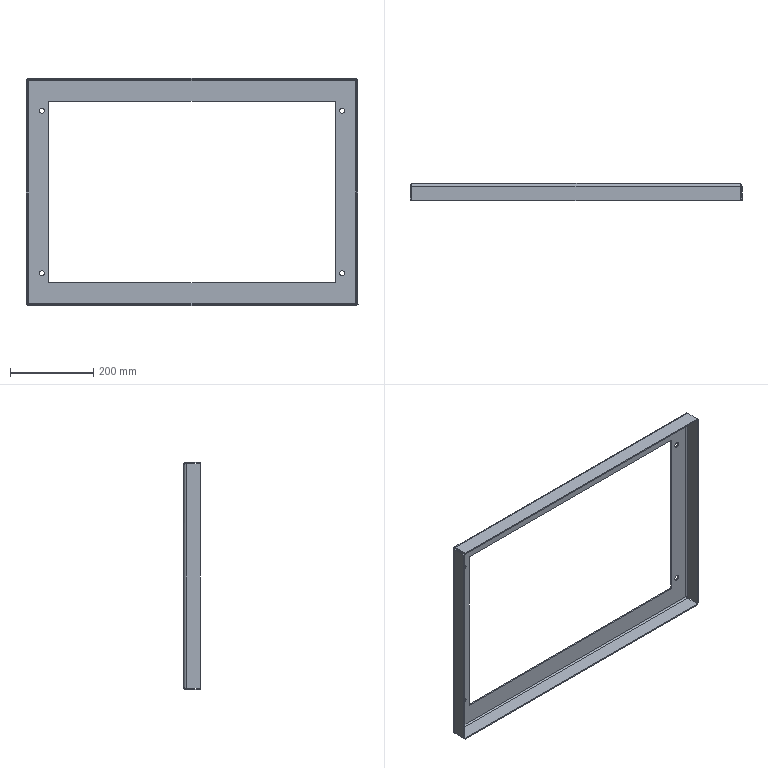Component | SolidWorks | StiffenerPlate-2 | 1 solid | 50 faces | volume 682149 mm3 | plane 26 | cylinder 16 | spline 8 | commonest cylinder face diameters 12.5 x8 7 x4 13 x4